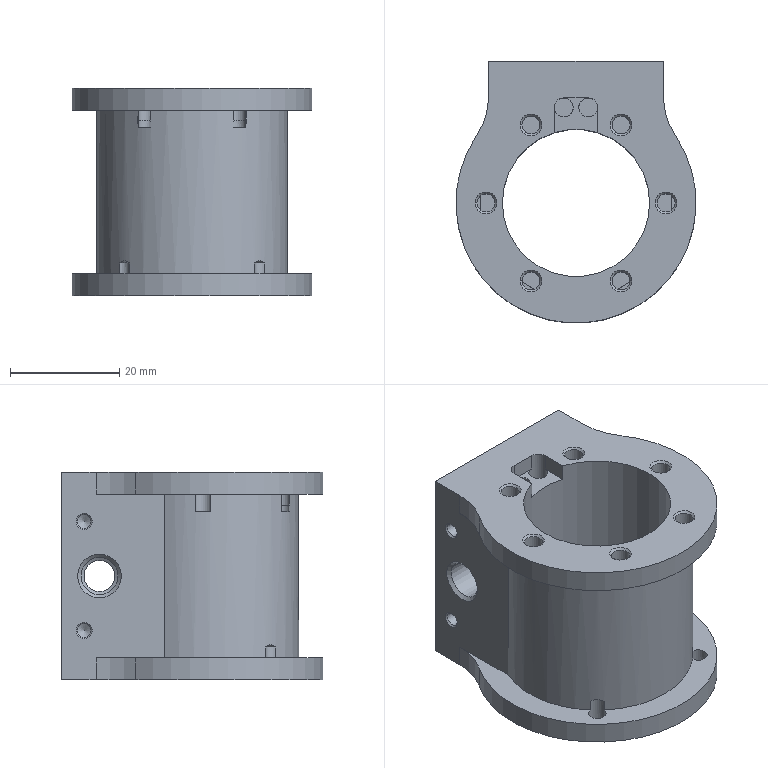Component | NX | UPPER_PISTON_CYLINDER | 1 solid | 126 faces | volume 27571 mm3 | cylinder 53 | plane 45 | cone 28 | commonest cylinder face diameters 3.3 x14 3.5 x8 2.5 x8 5 x4 26 x4 4 x4 4.024 x4 44 x2